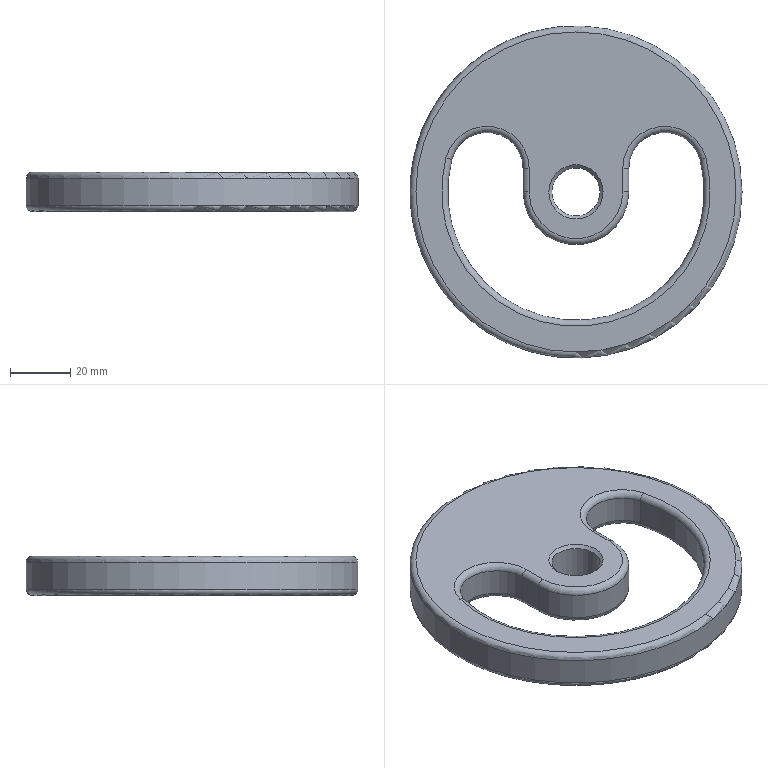Component | NX | HANDLE | 1 solid | 26 faces | volume 78271 mm3 | cylinder 10 | torus 10 | plane 4 | cone 2 | commonest cylinder face diameters 4 x4 24 x2 110 x1 85 x1 35 x1 16 x1